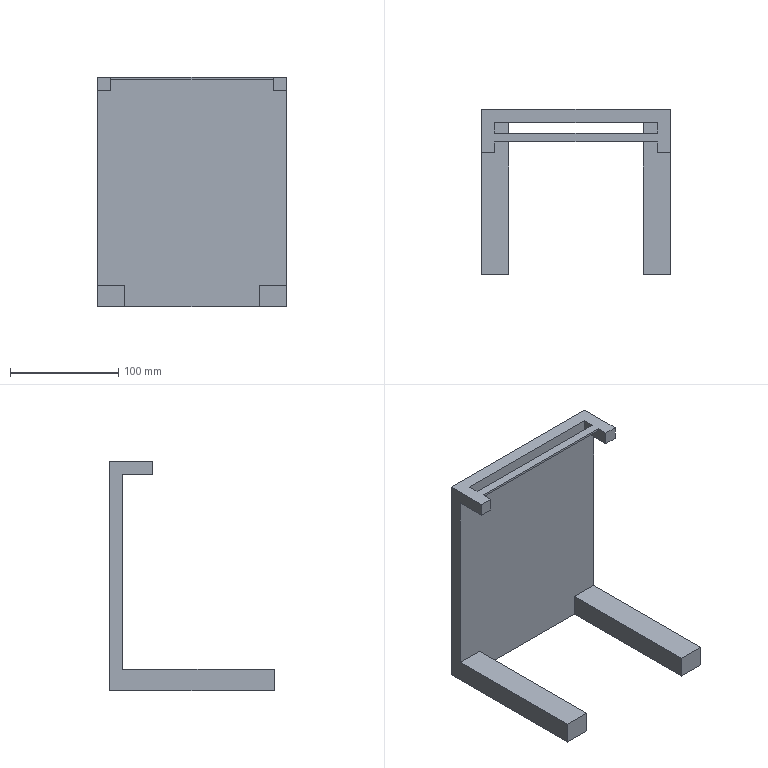Component | SolidWorks | SupportFrame-1 | 1 solid | 21 faces | box 174 x 152 x 212 mm | volume 593120 mm3 | plane 21
build123d program:
from build123d import *

# Parameters (mm, degrees)
SKETCH1_W             = 12
SKETCH1_H             = 12
BOSS_EXTRUDE1_DEPTH   = 40
BOSS_EXTRUDE1_2_DEPTH = 40
SKETCH2_W             = 12
SKETCH2_H             = 12
BOSS_EXTRUDE2_DEPTH   = 150
SKETCH3_W             = 150
SKETCH3_H             = 8
BOSS_EXTRUDE3_DEPTH   = 2
SKETCH4_W             = 174
SKETCH4_H             = 12
BOSS_EXTRUDE4_DEPTH   = 200
SKETCH5_W             = 25
SKETCH5_H             = 20
BOSS_EXTRUDE5_DEPTH   = 140


with BuildPart() as part:
    # Sketch1 → Boss-Extrude1 (new body)
    with BuildSketch(Plane.XY):
        with Locations((-299.265, -73.947)):
            Rectangle(SKETCH1_W, SKETCH1_H)
    extrude(amount=BOSS_EXTRUDE1_DEPTH)



with BuildPart() as body_2:
    # Sketch1 → Boss-Extrude1 2 (new body)
    with BuildSketch(Plane.XY):
        with Locations((-137.265, -73.947)):
            Rectangle(SKETCH1_W, SKETCH1_H)
    extrude(amount=BOSS_EXTRUDE1_2_DEPTH)


with BuildPart() as part_1:
    add(part.part)

    add(body_2.part)  # Boss-Extrude2 merges body 2
    # Sketch2 → Boss-Extrude2 (add)
    with BuildSketch(Plane.ZY.offset(143.265)):
        with Locations((34, -73.947)):
            Rectangle(SKETCH2_W, SKETCH2_H)
    extrude(amount=BOSS_EXTRUDE2_DEPTH)

    # Sketch3 → Boss-Extrude3 (add)
    with BuildSketch(Plane.XZ.offset(79.947)):
        with Locations((-218.265, 14)):
            Rectangle(SKETCH3_W, SKETCH3_H)
    extrude(amount=-BOSS_EXTRUDE3_DEPTH)

    # Sketch4 → Boss-Extrude4 (add)
    with BuildSketch(Plane(origin=(0, -67.947, 0), x_dir=(1, 0, 0), z_dir=(0, 1, 0))):
        with Locations((-218.265, -34)):
            Rectangle(SKETCH4_W, SKETCH4_H)
    extrude(amount=BOSS_EXTRUDE4_DEPTH)

    # Sketch5 → Boss-Extrude5 (add)
    with BuildSketch(Plane(origin=(0, 0, 28), x_dir=(-1, 0, 0), z_dir=(0, 0, -1))):
        with Locations((292.765, 122.053)):
            Rectangle(SKETCH5_W, SKETCH5_H)
        with Locations((143.765, 122.053)):
            Rectangle(SKETCH5_W, SKETCH5_H)
    extrude(amount=BOSS_EXTRUDE5_DEPTH)


solid = part_1.part

# Placed as in the assembly
solid = solid.moved(Location((-81.735, 110, 12.053), (-90, 0, 0)))
STEP:
#1=CARTESIAN_POINT('',(-8.386,5.433,-3.937));
#2=VERTEX_POINT('',#1);
#3=CARTESIAN_POINT('',(-9.37,5.433,-3.937));
#4=VERTEX_POINT('',#3);
#5=CARTESIAN_POINT('',(-8.386,5.433,-3.937));
#6=DIRECTION('',(-1.,0.,0.));
#7=VECTOR('',#6,39.37);
#8=LINE('',#5,#7);
#9=EDGE_CURVE('',#2,#4,#8,.T.);
#10=ORIENTED_EDGE('',*,*,#9,.F.);
#11=CARTESIAN_POINT('',(-8.386,5.433,3.15));
#12=VERTEX_POINT('',#11);
#13=CARTESIAN_POINT('',(-8.386,5.433,-4.724));
#14=DIRECTION('',(0.,0.,1.));
#15=VECTOR('',#14,39.37);
#16=LINE('',#13,#15);
#17=EDGE_CURVE('',#2,#12,#16,.T.);
#18=ORIENTED_EDGE('',*,*,#17,.T.);
#19=CARTESIAN_POINT('',(-8.858,5.433,3.15));
#20=VERTEX_POINT('',#19);
#21=CARTESIAN_POINT('',(-8.386,5.433,3.15));
#22=DIRECTION('',(-1.,0.,0.));
#23=VECTOR('',#22,39.37);
#24=LINE('',#21,#23);
#25=EDGE_CURVE('',#12,#20,#24,.T.);
#26=ORIENTED_EDGE('',*,*,#25,.T.);
#27=CARTESIAN_POINT('',(-8.858,5.433,3.622));
#28=VERTEX_POINT('',#27);
#29=CARTESIAN_POINT('',(-8.858,5.433,3.15));
#30=DIRECTION('',(0.,0.,1.));
#31=VECTOR('',#30,39.37);
#32=LINE('',#29,#31);
#33=EDGE_CURVE('',#20,#28,#32,.T.);
#34=ORIENTED_EDGE('',*,*,#33,.T.);
#35=CARTESIAN_POINT('',(-14.764,5.433,3.622));
#36=VERTEX_POINT('',#35);
#37=CARTESIAN_POINT('',(-15.432,5.433,3.622));
#38=DIRECTION('',(1.,0.,0.));
#39=VECTOR('',#38,39.37);
#40=LINE('',#37,#39);
#41=EDGE_CURVE('',#36,#28,#40,.T.);
#42=ORIENTED_EDGE('',*,*,#41,.F.);
#43=CARTESIAN_POINT('',(-14.764,5.433,3.15));
#44=VERTEX_POINT('',#43);
#45=CARTESIAN_POINT('',(-14.764,5.433,3.15));
#46=DIRECTION('',(0.,0.,1.));
#47=VECTOR('',#46,39.37);
#48=LINE('',#45,#47);
#49=EDGE_CURVE('',#44,#36,#48,.T.);
#50=ORIENTED_EDGE('',*,*,#49,.F.);
#51=CARTESIAN_POINT('',(-15.236,5.433,3.15));
#52=VERTEX_POINT('',#51);
#53=CARTESIAN_POINT('',(-8.386,5.433,3.15));
#54=DIRECTION('',(-1.,0.,0.));
#55=VECTOR('',#54,39.37);
#56=LINE('',#53,#55);
#57=EDGE_CURVE('',#44,#52,#56,.T.);
#58=ORIENTED_EDGE('',*,*,#57,.T.);
#59=CARTESIAN_POINT('',(-15.236,5.433,-3.937));
#60=VERTEX_POINT('',#59);
#61=CARTESIAN_POINT('',(-15.236,5.433,-4.724));
#62=DIRECTION('',(0.,0.,1.));
#63=VECTOR('',#62,39.37);
#64=LINE('',#61,#63);
#65=EDGE_CURVE('',#60,#52,#64,.T.);
#66=ORIENTED_EDGE('',*,*,#65,.F.);
#67=CARTESIAN_POINT('',(-14.252,5.433,-3.937));
#68=VERTEX_POINT('',#67);
#69=CARTESIAN_POINT('',(-15.236,5.433,-3.937));
#70=DIRECTION('',(-1.,0.,0.));
#71=VECTOR('',#70,39.37);
#72=LINE('',#69,#71);
#73=EDGE_CURVE('',#68,#60,#72,.T.);
#74=ORIENTED_EDGE('',*,*,#73,.F.);
#75=CARTESIAN_POINT('',(-14.252,5.433,-4.724));
#76=VERTEX_POINT('',#75);
#77=CARTESIAN_POINT('',(-14.252,5.433,-4.724));
#78=DIRECTION('',(0.,0.,1.));
#79=VECTOR('',#78,39.37);
#80=LINE('',#77,#79);
#81=EDGE_CURVE('',#76,#68,#80,.T.);
#82=ORIENTED_EDGE('',*,*,#81,.F.);
#83=CARTESIAN_POINT('',(-9.37,5.433,-4.724));
#84=VERTEX_POINT('',#83);
#85=CARTESIAN_POINT('',(-8.386,5.433,-4.724));
#86=DIRECTION('',(-1.,0.,0.));
#87=VECTOR('',#86,39.37);
#88=LINE('',#85,#87);
#89=EDGE_CURVE('',#84,#76,#88,.T.);
#90=ORIENTED_EDGE('',*,*,#89,.F.);
#91=CARTESIAN_POINT('',(-9.37,5.433,-4.724));
#92=DIRECTION('',(-0.,-0.,-1.));
#93=VECTOR('',#92,39.37);
#94=LINE('',#91,#93);
#95=EDGE_CURVE('',#4,#84,#94,.T.);
#96=ORIENTED_EDGE('',*,*,#95,.F.);
#97=EDGE_LOOP('',(#10,#18,#26,#34,#42,#50,#58,#66,#74,#82,#90,#96));
#98=FACE_OUTER_BOUND('',#97,.T.);
#99=CARTESIAN_POINT('',(-15.432,5.433,3.15));
#100=DIRECTION('',(0.,1.,-0.));
#101=DIRECTION('',(0.,0.,1.));
#102=AXIS2_PLACEMENT_3D('',#99,#100,#101);
#103=PLANE('',#102);
#104=ADVANCED_FACE('',(#98),#103,.F.);
#105=ORIENTED_EDGE('',*,*,#25,.F.);
#106=CARTESIAN_POINT('',(-8.386,4.331,3.15));
#107=VERTEX_POINT('',#106);
#108=CARTESIAN_POINT('',(-8.386,5.906,3.15));
#109=DIRECTION('',(0.,-1.,0.));
#110=VECTOR('',#109,39.37);
#111=LINE('',#108,#110);
#112=EDGE_CURVE('',#12,#107,#111,.T.);
#113=ORIENTED_EDGE('',*,*,#112,.T.);
#114=CARTESIAN_POINT('',(-8.858,4.331,3.15));
#115=VERTEX_POINT('',#114);
#116=CARTESIAN_POINT('',(-8.858,4.331,3.15));
#117=DIRECTION('',(-1.,0.,0.));
#118=VECTOR('',#117,39.37);
#119=LINE('',#116,#118);
#120=EDGE_CURVE('',#107,#115,#119,.T.);
#121=ORIENTED_EDGE('',*,*,#120,.T.);
#122=CARTESIAN_POINT('',(-8.858,5.906,3.15));
#123=DIRECTION('',(0.,-1.,0.));
#124=VECTOR('',#123,39.37);
#125=LINE('',#122,#124);
#126=EDGE_CURVE('',#20,#115,#125,.T.);
#127=ORIENTED_EDGE('',*,*,#126,.F.);
#128=EDGE_LOOP('',(#105,#113,#121,#127));
#129=FACE_OUTER_BOUND('',#128,.T.);
#130=CARTESIAN_POINT('',(-15.236,5.906,3.15));
#131=DIRECTION('',(0.,0.,1.));
#132=DIRECTION('',(0.,-1.,0.));
#133=AXIS2_PLACEMENT_3D('',#130,#131,#132);
#134=PLANE('',#133);
#135=ADVANCED_FACE('',(#129),#134,.F.);
#136=ORIENTED_EDGE('',*,*,#57,.F.);
#137=CARTESIAN_POINT('',(-14.764,4.331,3.15));
#138=VERTEX_POINT('',#137);
#139=CARTESIAN_POINT('',(-14.764,5.906,3.15));
#140=DIRECTION('',(0.,-1.,0.));
#141=VECTOR('',#140,39.37);
#142=LINE('',#139,#141);
#143=EDGE_CURVE('',#44,#138,#142,.T.);
#144=ORIENTED_EDGE('',*,*,#143,.T.);
#145=CARTESIAN_POINT('',(-15.236,4.331,3.15));
#146=VERTEX_POINT('',#145);
#147=CARTESIAN_POINT('',(-15.236,4.331,3.15));
#148=DIRECTION('',(-1.,0.,0.));
#149=VECTOR('',#148,39.37);
#150=LINE('',#147,#149);
#151=EDGE_CURVE('',#138,#146,#150,.T.);
#152=ORIENTED_EDGE('',*,*,#151,.T.);
#153=CARTESIAN_POINT('',(-15.236,5.906,3.15));
#154=DIRECTION('',(0.,-1.,0.));
#155=VECTOR('',#154,39.37);
#156=LINE('',#153,#155);
#157=EDGE_CURVE('',#52,#146,#156,.T.);
#158=ORIENTED_EDGE('',*,*,#157,.F.);
#159=EDGE_LOOP('',(#136,#144,#152,#158));
#160=FACE_OUTER_BOUND('',#159,.T.);
#161=CARTESIAN_POINT('',(-15.236,5.906,3.15));
#162=DIRECTION('',(0.,0.,1.));
#163=DIRECTION('',(0.,-1.,0.));
#164=AXIS2_PLACEMENT_3D('',#161,#162,#163);
#165=PLANE('',#164);
#166=ADVANCED_FACE('',(#160),#165,.F.);
#167=CARTESIAN_POINT('',(-15.236,4.331,3.622));
#168=VERTEX_POINT('',#167);
#169=CARTESIAN_POINT('',(-15.236,4.331,3.622));
#170=DIRECTION('',(0.,0.,1.));
#171=VECTOR('',#170,39.37);
#172=LINE('',#169,#171);
#173=EDGE_CURVE('',#146,#168,#172,.T.);
#174=ORIENTED_EDGE('',*,*,#173,.T.);
#175=CARTESIAN_POINT('',(-15.236,5.906,3.622));
#176=VERTEX_POINT('',#175);
#177=CARTESIAN_POINT('',(-15.236,5.906,3.622));
#178=DIRECTION('',(0.,-1.,0.));
#179=VECTOR('',#178,39.37);
#180=LINE('',#177,#179);
#181=EDGE_CURVE('',#176,#168,#180,.T.);
#182=ORIENTED_EDGE('',*,*,#181,.F.);
#183=CARTESIAN_POINT('',(-15.236,5.906,-4.724));
#184=VERTEX_POINT('',#183);
#185=CARTESIAN_POINT('',(-15.236,5.906,3.622));
#186=DIRECTION('',(0.,0.,1.));
#187=VECTOR('',#186,39.37);
#188=LINE('',#185,#187);
#189=EDGE_CURVE('',#184,#176,#188,.T.);
#190=ORIENTED_EDGE('',*,*,#189,.F.);
#191=CARTESIAN_POINT('',(-15.236,-0.07874,-4.724));
#192=VERTEX_POINT('',#191);
#193=CARTESIAN_POINT('',(-15.236,5.906,-4.724));
#194=DIRECTION('',(0.,1.,0.));
#195=VECTOR('',#194,39.37);
#196=LINE('',#193,#195);
#197=EDGE_CURVE('',#192,#184,#196,.T.);
#198=ORIENTED_EDGE('',*,*,#197,.F.);
#199=CARTESIAN_POINT('',(-15.236,-0.07874,-3.937));
#200=VERTEX_POINT('',#199);
#201=CARTESIAN_POINT('',(-15.236,-0.07874,-4.724));
#202=DIRECTION('',(0.,-0.,-1.));
#203=VECTOR('',#202,39.37);
#204=LINE('',#201,#203);
#205=EDGE_CURVE('',#200,#192,#204,.T.);
#206=ORIENTED_EDGE('',*,*,#205,.F.);
#207=CARTESIAN_POINT('',(-15.236,-0.07874,-3.937));
#208=DIRECTION('',(0.,1.,-0.));
#209=VECTOR('',#208,39.37);
#210=LINE('',#207,#209);
#211=EDGE_CURVE('',#200,#60,#210,.T.);
#212=ORIENTED_EDGE('',*,*,#211,.T.);
#213=ORIENTED_EDGE('',*,*,#65,.T.);
#214=ORIENTED_EDGE('',*,*,#157,.T.);
#215=EDGE_LOOP('',(#174,#182,#190,#198,#206,#212,#213,#214));
#216=FACE_OUTER_BOUND('',#215,.T.);
#217=CARTESIAN_POINT('',(-15.236,5.906,3.622));
#218=DIRECTION('',(1.,0.,0.));
#219=DIRECTION('',(0.,-1.,0.));
#220=AXIS2_PLACEMENT_3D('',#217,#218,#219);
#221=PLANE('',#220);
#222=ADVANCED_FACE('',(#216),#221,.F.);
#223=CARTESIAN_POINT('',(-14.764,4.724,3.622));
#224=VERTEX_POINT('',#223);
#225=CARTESIAN_POINT('',(-14.764,4.331,3.622));
#226=VERTEX_POINT('',#225);
#227=CARTESIAN_POINT('',(-14.764,5.906,3.622));
#228=DIRECTION('',(0.,-1.,0.));
#229=VECTOR('',#228,39.37);
#230=LINE('',#227,#229);
#231=EDGE_CURVE('',#224,#226,#230,.T.);
#232=ORIENTED_EDGE('',*,*,#231,.F.);
#233=CARTESIAN_POINT('',(-8.858,4.724,3.622));
#234=VERTEX_POINT('',#233);
#235=CARTESIAN_POINT('',(-14.764,4.724,3.622));
#236=DIRECTION('',(1.,0.,0.));
#237=VECTOR('',#236,39.37);
#238=LINE('',#235,#237);
#239=EDGE_CURVE('',#224,#234,#238,.T.);
#240=ORIENTED_EDGE('',*,*,#239,.T.);
#241=CARTESIAN_POINT('',(-8.858,4.331,3.622));
#242=VERTEX_POINT('',#241);
#243=CARTESIAN_POINT('',(-8.858,5.906,3.622));
#244=DIRECTION('',(0.,-1.,0.));
#245=VECTOR('',#244,39.37);
#246=LINE('',#243,#245);
#247=EDGE_CURVE('',#234,#242,#246,.T.);
#248=ORIENTED_EDGE('',*,*,#247,.T.);
#249=CARTESIAN_POINT('',(-8.386,4.331,3.622));
#250=VERTEX_POINT('',#249);
#251=CARTESIAN_POINT('',(-8.858,4.331,3.622));
#252=DIRECTION('',(1.,0.,0.));
#253=VECTOR('',#252,39.37);
#254=LINE('',#251,#253);
#255=EDGE_CURVE('',#242,#250,#254,.T.);
#256=ORIENTED_EDGE('',*,*,#255,.T.);
#257=CARTESIAN_POINT('',(-8.386,5.906,3.622));
#258=VERTEX_POINT('',#257);
#259=CARTESIAN_POINT('',(-8.386,5.906,3.622));
#260=DIRECTION('',(0.,-1.,0.));
#261=VECTOR('',#260,39.37);
#262=LINE('',#259,#261);
#263=EDGE_CURVE('',#258,#250,#262,.T.);
#264=ORIENTED_EDGE('',*,*,#263,.F.);
#265=CARTESIAN_POINT('',(-15.236,5.906,3.622));
#266=DIRECTION('',(1.,0.,0.));
#267=VECTOR('',#266,39.37);
#268=LINE('',#265,#267);
#269=EDGE_CURVE('',#176,#258,#268,.T.);
#270=ORIENTED_EDGE('',*,*,#269,.F.);
#271=ORIENTED_EDGE('',*,*,#181,.T.);
#272=CARTESIAN_POINT('',(-15.236,4.331,3.622));
#273=DIRECTION('',(1.,0.,0.));
#274=VECTOR('',#273,39.37);
#275=LINE('',#272,#274);
#276=EDGE_CURVE('',#168,#226,#275,.T.);
#277=ORIENTED_EDGE('',*,*,#276,.T.);
#278=EDGE_LOOP('',(#232,#240,#248,#256,#264,#270,#271,#277));
#279=FACE_OUTER_BOUND('',#278,.T.);
#280=CARTESIAN_POINT('',(-8.858,5.039,3.622));
#281=VERTEX_POINT('',#280);
#282=CARTESIAN_POINT('',(-14.764,5.039,3.622));
#283=VERTEX_POINT('',#282);
#284=CARTESIAN_POINT('',(-14.764,5.039,3.622));
#285=DIRECTION('',(-1.,0.,0.));
#286=VECTOR('',#285,39.37);
#287=LINE('',#284,#286);
#288=EDGE_CURVE('',#281,#283,#287,.T.);
#289=ORIENTED_EDGE('',*,*,#288,.T.);
#290=CARTESIAN_POINT('',(-14.764,5.906,3.622));
#291=DIRECTION('',(0.,-1.,0.));
#292=VECTOR('',#291,39.37);
#293=LINE('',#290,#292);
#294=EDGE_CURVE('',#36,#283,#293,.T.);
#295=ORIENTED_EDGE('',*,*,#294,.F.);
#296=ORIENTED_EDGE('',*,*,#41,.T.);
#297=CARTESIAN_POINT('',(-8.858,5.906,3.622));
#298=DIRECTION('',(0.,-1.,0.));
#299=VECTOR('',#298,39.37);
#300=LINE('',#297,#299);
#301=EDGE_CURVE('',#28,#281,#300,.T.);
#302=ORIENTED_EDGE('',*,*,#301,.T.);
#303=EDGE_LOOP('',(#289,#295,#296,#302));
#304=FACE_BOUND('',#303,.T.);
#305=CARTESIAN_POINT('',(-15.236,5.906,3.622));
#306=DIRECTION('',(0.,0.,-1.));
#307=DIRECTION('',(0.,1.,0.));
#308=AXIS2_PLACEMENT_3D('',#305,#306,#307);
#309=PLANE('',#308);
#310=ADVANCED_FACE('',(#279,#304),#309,.F.);
#311=ORIENTED_EDGE('',*,*,#294,.T.);
#312=CARTESIAN_POINT('',(-14.764,5.039,3.543));
#313=VERTEX_POINT('',#312);
#314=CARTESIAN_POINT('',(-14.764,5.039,3.543));
#315=DIRECTION('',(0.,0.,1.));
#316=VECTOR('',#315,39.37);
#317=LINE('',#314,#316);
#318=EDGE_CURVE('',#313,#283,#317,.T.);
#319=ORIENTED_EDGE('',*,*,#318,.F.);
#320=CARTESIAN_POINT('',(-14.764,4.724,3.543));
#321=VERTEX_POINT('',#320);
#322=CARTESIAN_POINT('',(-14.764,5.039,3.543));
#323=DIRECTION('',(0.,-1.,0.));
#324=VECTOR('',#323,39.37);
#325=LINE('',#322,#324);
#326=EDGE_CURVE('',#313,#321,#325,.T.);
#327=ORIENTED_EDGE('',*,*,#326,.T.);
#328=CARTESIAN_POINT('',(-14.764,4.724,3.543));
#329=DIRECTION('',(0.,0.,1.));
#330=VECTOR('',#329,39.37);
#331=LINE('',#328,#330);
#332=EDGE_CURVE('',#321,#224,#331,.T.);
#333=ORIENTED_EDGE('',*,*,#332,.T.);
#334=ORIENTED_EDGE('',*,*,#231,.T.);
#335=CARTESIAN_POINT('',(-14.764,4.331,3.622));
#336=DIRECTION('',(0.,0.,-1.));
#337=VECTOR('',#336,39.37);
#338=LINE('',#335,#337);
#339=EDGE_CURVE('',#226,#138,#338,.T.);
#340=ORIENTED_EDGE('',*,*,#339,.T.);
#341=ORIENTED_EDGE('',*,*,#143,.F.);
#342=ORIENTED_EDGE('',*,*,#49,.T.);
#343=EDGE_LOOP('',(#311,#319,#327,#333,#334,#340,#341,#342));
#344=FACE_OUTER_BOUND('',#343,.T.);
#345=CARTESIAN_POINT('',(-14.764,5.906,3.622));
#346=DIRECTION('',(-1.,0.,0.));
#347=DIRECTION('',(0.,1.,0.));
#348=AXIS2_PLACEMENT_3D('',#345,#346,#347);
#349=PLANE('',#348);
#350=ADVANCED_FACE('',(#344),#349,.F.);
#351=ORIENTED_EDGE('',*,*,#189,.T.);
#352=ORIENTED_EDGE('',*,*,#269,.T.);
#353=CARTESIAN_POINT('',(-8.386,5.906,-4.724));
#354=VERTEX_POINT('',#353);
#355=CARTESIAN_POINT('',(-8.386,5.906,3.622));
#356=DIRECTION('',(0.,0.,-1.));
#357=VECTOR('',#356,39.37);
#358=LINE('',#355,#357);
#359=EDGE_CURVE('',#258,#354,#358,.T.);
#360=ORIENTED_EDGE('',*,*,#359,.T.);
#361=CARTESIAN_POINT('',(-8.386,5.906,-4.724));
#362=DIRECTION('',(1.,0.,0.));
#363=VECTOR('',#362,39.37);
#364=LINE('',#361,#363);
#365=EDGE_CURVE('',#184,#354,#364,.T.);
#366=ORIENTED_EDGE('',*,*,#365,.F.);
#367=EDGE_LOOP('',(#351,#352,#360,#366));
#368=FACE_OUTER_BOUND('',#367,.T.);
#369=CARTESIAN_POINT('',(-3.218,5.906,0.4745));
#370=DIRECTION('',(0.,-1.,0.));
#371=DIRECTION('',(-1.,0.,0.));
#372=AXIS2_PLACEMENT_3D('',#369,#370,#371);
#373=PLANE('',#372);
#374=ADVANCED_FACE('',(#368),#373,.F.);
#375=ORIENTED_EDGE('',*,*,#173,.F.);
#376=ORIENTED_EDGE('',*,*,#151,.F.);
#377=ORIENTED_EDGE('',*,*,#339,.F.);
#378=ORIENTED_EDGE('',*,*,#276,.F.);
#379=EDGE_LOOP('',(#375,#376,#377,#378));
#380=FACE_OUTER_BOUND('',#379,.T.);
#381=CARTESIAN_POINT('',(-3.218,4.331,0.4745));
#382=DIRECTION('',(0.,-1.,0.));
#383=DIRECTION('',(-1.,0.,0.));
#384=AXIS2_PLACEMENT_3D('',#381,#382,#383);
#385=PLANE('',#384);
#386=ADVANCED_FACE('',(#380),#385,.T.);
#387=CARTESIAN_POINT('',(-8.858,4.724,3.543));
#388=VERTEX_POINT('',#387);
#389=CARTESIAN_POINT('',(-8.858,5.039,3.543));
#390=VERTEX_POINT('',#389);
#391=CARTESIAN_POINT('',(-8.858,5.039,3.543));
#392=DIRECTION('',(0.,1.,0.));
#393=VECTOR('',#392,39.37);
#394=LINE('',#391,#393);
#395=EDGE_CURVE('',#388,#390,#394,.T.);
#396=ORIENTED_EDGE('',*,*,#395,.T.);
#397=CARTESIAN_POINT('',(-8.858,5.039,3.543));
#398=DIRECTION('',(0.,0.,1.));
#399=VECTOR('',#398,39.37);
#400=LINE('',#397,#399);
#401=EDGE_CURVE('',#390,#281,#400,.T.);
#402=ORIENTED_EDGE('',*,*,#401,.T.);
#403=ORIENTED_EDGE('',*,*,#301,.F.);
#404=ORIENTED_EDGE('',*,*,#33,.F.);
#405=ORIENTED_EDGE('',*,*,#126,.T.);
#406=CARTESIAN_POINT('',(-8.858,4.331,3.622));
#407=DIRECTION('',(0.,0.,1.));
#408=VECTOR('',#407,39.37);
#409=LINE('',#406,#408);
#410=EDGE_CURVE('',#115,#242,#409,.T.);
#411=ORIENTED_EDGE('',*,*,#410,.T.);
#412=ORIENTED_EDGE('',*,*,#247,.F.);
#413=CARTESIAN_POINT('',(-8.858,4.724,3.543));
#414=DIRECTION('',(0.,0.,1.));
#415=VECTOR('',#414,39.37);
#416=LINE('',#413,#415);
#417=EDGE_CURVE('',#388,#234,#416,.T.);
#418=ORIENTED_EDGE('',*,*,#417,.F.);
#419=EDGE_LOOP('',(#396,#402,#403,#404,#405,#411,#412,#418));
#420=FACE_OUTER_BOUND('',#419,.T.);
#421=CARTESIAN_POINT('',(-8.858,5.906,3.622));
#422=DIRECTION('',(1.,0.,0.));
#423=DIRECTION('',(0.,-1.,0.));
#424=AXIS2_PLACEMENT_3D('',#421,#422,#423);
#425=PLANE('',#424);
#426=ADVANCED_FACE('',(#420),#425,.F.);
#427=CARTESIAN_POINT('',(-8.386,4.331,3.622));
#428=DIRECTION('',(0.,0.,-1.));
#429=VECTOR('',#428,39.37);
#430=LINE('',#427,#429);
#431=EDGE_CURVE('',#250,#107,#430,.T.);
#432=ORIENTED_EDGE('',*,*,#431,.T.);
#433=ORIENTED_EDGE('',*,*,#112,.F.);
#434=ORIENTED_EDGE('',*,*,#17,.F.);
#435=CARTESIAN_POINT('',(-8.386,-0.07874,-3.937));
#436=VERTEX_POINT('',#435);
#437=CARTESIAN_POINT('',(-8.386,-0.07874,-3.937));
#438=DIRECTION('',(0.,1.,-0.));
#439=VECTOR('',#438,39.37);
#440=LINE('',#437,#439);
#441=EDGE_CURVE('',#436,#2,#440,.T.);
#442=ORIENTED_EDGE('',*,*,#441,.F.);
#443=CARTESIAN_POINT('',(-8.386,-0.07874,-4.724));
#444=VERTEX_POINT('',#443);
#445=CARTESIAN_POINT('',(-8.386,-0.07874,-4.724));
#446=DIRECTION('',(0.,0.,1.));
#447=VECTOR('',#446,39.37);
#448=LINE('',#445,#447);
#449=EDGE_CURVE('',#444,#436,#448,.T.);
#450=ORIENTED_EDGE('',*,*,#449,.F.);
#451=CARTESIAN_POINT('',(-8.386,5.906,-4.724));
#452=DIRECTION('',(0.,-1.,0.));
#453=VECTOR('',#452,39.37);
#454=LINE('',#451,#453);
#455=EDGE_CURVE('',#354,#444,#454,.T.);
#456=ORIENTED_EDGE('',*,*,#455,.F.);
#457=ORIENTED_EDGE('',*,*,#359,.F.);
#458=ORIENTED_EDGE('',*,*,#263,.T.);
#459=EDGE_LOOP('',(#432,#433,#434,#442,#450,#456,#457,#458));
#460=FACE_OUTER_BOUND('',#459,.T.);
#461=CARTESIAN_POINT('',(-8.386,5.906,3.622));
#462=DIRECTION('',(-1.,0.,0.));
#463=DIRECTION('',(0.,1.,0.));
#464=AXIS2_PLACEMENT_3D('',#461,#462,#463);
#465=PLANE('',#464);
#466=ADVANCED_FACE('',(#460),#465,.F.);
#467=ORIENTED_EDGE('',*,*,#410,.F.);
#468=ORIENTED_EDGE('',*,*,#120,.F.);
#469=ORIENTED_EDGE('',*,*,#431,.F.);
#470=ORIENTED_EDGE('',*,*,#255,.F.);
#471=EDGE_LOOP('',(#467,#468,#469,#470));
#472=FACE_OUTER_BOUND('',#471,.T.);
#473=CARTESIAN_POINT('',(-3.218,4.331,0.4745));
#474=DIRECTION('',(0.,-1.,0.));
#475=DIRECTION('',(-1.,0.,0.));
#476=AXIS2_PLACEMENT_3D('',#473,#474,#475);
#477=PLANE('',#476);
#478=ADVANCED_FACE('',(#472),#477,.T.);
#479=ORIENTED_EDGE('',*,*,#288,.F.);
#480=ORIENTED_EDGE('',*,*,#401,.F.);
#481=CARTESIAN_POINT('',(-14.764,5.039,3.543));
#482=DIRECTION('',(-1.,0.,0.));
#483=VECTOR('',#482,39.37);
#484=LINE('',#481,#483);
#485=EDGE_CURVE('',#390,#313,#484,.T.);
#486=ORIENTED_EDGE('',*,*,#485,.T.);
#487=ORIENTED_EDGE('',*,*,#318,.T.);
#488=EDGE_LOOP('',(#479,#480,#486,#487));
#489=FACE_OUTER_BOUND('',#488,.T.);
#490=CARTESIAN_POINT('',(-14.764,5.039,3.543));
#491=DIRECTION('',(0.,1.,0.));
#492=DIRECTION('',(1.,0.,0.));
#493=AXIS2_PLACEMENT_3D('',#490,#491,#492);
#494=PLANE('',#493);
#495=ADVANCED_FACE('',(#489),#494,.T.);
#496=ORIENTED_EDGE('',*,*,#239,.F.);
#497=ORIENTED_EDGE('',*,*,#332,.F.);
#498=CARTESIAN_POINT('',(-14.764,4.724,3.543));
#499=DIRECTION('',(1.,0.,0.));
#500=VECTOR('',#499,39.37);
#501=LINE('',#498,#500);
#502=EDGE_CURVE('',#321,#388,#501,.T.);
#503=ORIENTED_EDGE('',*,*,#502,.T.);
#504=ORIENTED_EDGE('',*,*,#417,.T.);
#505=EDGE_LOOP('',(#496,#497,#503,#504));
#506=FACE_OUTER_BOUND('',#505,.T.);
#507=CARTESIAN_POINT('',(-14.764,4.724,3.543));
#508=DIRECTION('',(0.,-1.,0.));
#509=DIRECTION('',(-1.,0.,0.));
#510=AXIS2_PLACEMENT_3D('',#507,#508,#509);
#511=PLANE('',#510);
#512=ADVANCED_FACE('',(#506),#511,.T.);
#513=ORIENTED_EDGE('',*,*,#326,.F.);
#514=ORIENTED_EDGE('',*,*,#485,.F.);
#515=ORIENTED_EDGE('',*,*,#395,.F.);
#516=ORIENTED_EDGE('',*,*,#502,.F.);
#517=EDGE_LOOP('',(#513,#514,#515,#516));
#518=FACE_OUTER_BOUND('',#517,.T.);
#519=CARTESIAN_POINT('',(-3.218,4.331,3.543));
#520=DIRECTION('',(0.,0.,1.));
#521=DIRECTION('',(0.,-1.,0.));
#522=AXIS2_PLACEMENT_3D('',#519,#520,#521);
#523=PLANE('',#522);
#524=ADVANCED_FACE('',(#518),#523,.F.);
#525=ORIENTED_EDGE('',*,*,#455,.T.);
#526=CARTESIAN_POINT('',(-9.37,-0.07874,-4.724));
#527=VERTEX_POINT('',#526);
#528=CARTESIAN_POINT('',(-8.386,-0.07874,-4.724));
#529=DIRECTION('',(1.,0.,0.));
#530=VECTOR('',#529,39.37);
#531=LINE('',#528,#530);
#532=EDGE_CURVE('',#527,#444,#531,.T.);
#533=ORIENTED_EDGE('',*,*,#532,.F.);
#534=CARTESIAN_POINT('',(-9.37,-0.07874,-4.724));
#535=DIRECTION('',(0.,1.,-0.));
#536=VECTOR('',#535,39.37);
#537=LINE('',#534,#536);
#538=EDGE_CURVE('',#527,#84,#537,.T.);
#539=ORIENTED_EDGE('',*,*,#538,.T.);
#540=ORIENTED_EDGE('',*,*,#89,.T.);
#541=CARTESIAN_POINT('',(-14.252,-0.07874,-4.724));
#542=VERTEX_POINT('',#541);
#543=CARTESIAN_POINT('',(-14.252,-0.07874,-4.724));
#544=DIRECTION('',(0.,1.,-0.));
#545=VECTOR('',#544,39.37);
#546=LINE('',#543,#545);
#547=EDGE_CURVE('',#542,#76,#546,.T.);
#548=ORIENTED_EDGE('',*,*,#547,.F.);
#549=CARTESIAN_POINT('',(-15.236,-0.07874,-4.724));
#550=DIRECTION('',(1.,0.,0.));
#551=VECTOR('',#550,39.37);
#552=LINE('',#549,#551);
#553=EDGE_CURVE('',#192,#542,#552,.T.);
#554=ORIENTED_EDGE('',*,*,#553,.F.);
#555=ORIENTED_EDGE('',*,*,#197,.T.);
#556=ORIENTED_EDGE('',*,*,#365,.T.);
#557=EDGE_LOOP('',(#525,#533,#539,#540,#548,#554,#555,#556));
#558=FACE_OUTER_BOUND('',#557,.T.);
#559=CARTESIAN_POINT('',(-3.218,4.331,-4.724));
#560=DIRECTION('',(0.,0.,-1.));
#561=DIRECTION('',(0.,1.,0.));
#562=AXIS2_PLACEMENT_3D('',#559,#560,#561);
#563=PLANE('',#562);
#564=ADVANCED_FACE('',(#558),#563,.T.);
#565=ORIENTED_EDGE('',*,*,#81,.T.);
#566=CARTESIAN_POINT('',(-14.252,-0.07874,-3.937));
#567=VERTEX_POINT('',#566);
#568=CARTESIAN_POINT('',(-14.252,-0.07874,-3.937));
#569=DIRECTION('',(0.,1.,-0.));
#570=VECTOR('',#569,39.37);
#571=LINE('',#568,#570);
#572=EDGE_CURVE('',#567,#68,#571,.T.);
#573=ORIENTED_EDGE('',*,*,#572,.F.);
#574=CARTESIAN_POINT('',(-14.252,-0.07874,-4.724));
#575=DIRECTION('',(0.,0.,1.));
#576=VECTOR('',#575,39.37);
#577=LINE('',#574,#576);
#578=EDGE_CURVE('',#542,#567,#577,.T.);
#579=ORIENTED_EDGE('',*,*,#578,.F.);
#580=ORIENTED_EDGE('',*,*,#547,.T.);
#581=EDGE_LOOP('',(#565,#573,#579,#580));
#582=FACE_OUTER_BOUND('',#581,.T.);
#583=CARTESIAN_POINT('',(-14.252,-0.07874,-4.724));
#584=DIRECTION('',(-1.,0.,0.));
#585=DIRECTION('',(0.,1.,0.));
#586=AXIS2_PLACEMENT_3D('',#583,#584,#585);
#587=PLANE('',#586);
#588=ADVANCED_FACE('',(#582),#587,.F.);
#589=ORIENTED_EDGE('',*,*,#73,.T.);
#590=ORIENTED_EDGE('',*,*,#211,.F.);
#591=CARTESIAN_POINT('',(-15.236,-0.07874,-3.937));
#592=DIRECTION('',(-1.,0.,0.));
#593=VECTOR('',#592,39.37);
#594=LINE('',#591,#593);
#595=EDGE_CURVE('',#567,#200,#594,.T.);
#596=ORIENTED_EDGE('',*,*,#595,.F.);
#597=ORIENTED_EDGE('',*,*,#572,.T.);
#598=EDGE_LOOP('',(#589,#590,#596,#597));
#599=FACE_OUTER_BOUND('',#598,.T.);
#600=CARTESIAN_POINT('',(-15.236,-0.07874,-3.937));
#601=DIRECTION('',(0.,-0.,-1.));
#602=DIRECTION('',(0.,1.,-0.));
#603=AXIS2_PLACEMENT_3D('',#600,#601,#602);
#604=PLANE('',#603);
#605=ADVANCED_FACE('',(#599),#604,.F.);
#606=ORIENTED_EDGE('',*,*,#205,.T.);
#607=ORIENTED_EDGE('',*,*,#553,.T.);
#608=ORIENTED_EDGE('',*,*,#578,.T.);
#609=ORIENTED_EDGE('',*,*,#595,.T.);
#610=EDGE_LOOP('',(#606,#607,#608,#609));
#611=FACE_OUTER_BOUND('',#610,.T.);
#612=CARTESIAN_POINT('',(-3.218,-0.07874,0.4745));
#613=DIRECTION('',(0.,1.,-0.));
#614=DIRECTION('',(0.,0.,1.));
#615=AXIS2_PLACEMENT_3D('',#612,#613,#614);
#616=PLANE('',#615);
#617=ADVANCED_FACE('',(#611),#616,.F.);
#618=ORIENTED_EDGE('',*,*,#9,.T.);
#619=CARTESIAN_POINT('',(-9.37,-0.07874,-3.937));
#620=VERTEX_POINT('',#619);
#621=CARTESIAN_POINT('',(-9.37,-0.07874,-3.937));
#622=DIRECTION('',(0.,1.,-0.));
#623=VECTOR('',#622,39.37);
#624=LINE('',#621,#623);
#625=EDGE_CURVE('',#620,#4,#624,.T.);
#626=ORIENTED_EDGE('',*,*,#625,.F.);
#627=CARTESIAN_POINT('',(-8.386,-0.07874,-3.937));
#628=DIRECTION('',(-1.,0.,0.));
#629=VECTOR('',#628,39.37);
#630=LINE('',#627,#629);
#631=EDGE_CURVE('',#436,#620,#630,.T.);
#632=ORIENTED_EDGE('',*,*,#631,.F.);
#633=ORIENTED_EDGE('',*,*,#441,.T.);
#634=EDGE_LOOP('',(#618,#626,#632,#633));
#635=FACE_OUTER_BOUND('',#634,.T.);
#636=CARTESIAN_POINT('',(-8.386,-0.07874,-3.937));
#637=DIRECTION('',(0.,-0.,-1.));
#638=DIRECTION('',(0.,1.,-0.));
#639=AXIS2_PLACEMENT_3D('',#636,#637,#638);
#640=PLANE('',#639);
#641=ADVANCED_FACE('',(#635),#640,.F.);
#642=ORIENTED_EDGE('',*,*,#95,.T.);
#643=ORIENTED_EDGE('',*,*,#538,.F.);
#644=CARTESIAN_POINT('',(-9.37,-0.07874,-4.724));
#645=DIRECTION('',(-0.,-0.,-1.));
#646=VECTOR('',#645,39.37);
#647=LINE('',#644,#646);
#648=EDGE_CURVE('',#620,#527,#647,.T.);
#649=ORIENTED_EDGE('',*,*,#648,.F.);
#650=ORIENTED_EDGE('',*,*,#625,.T.);
#651=EDGE_LOOP('',(#642,#643,#649,#650));
#652=FACE_OUTER_BOUND('',#651,.T.);
#653=CARTESIAN_POINT('',(-9.37,-0.07874,-4.724));
#654=DIRECTION('',(1.,-0.,-0.));
#655=DIRECTION('',(-0.,0.,-1.));
#656=AXIS2_PLACEMENT_3D('',#653,#654,#655);
#657=PLANE('',#656);
#658=ADVANCED_FACE('',(#652),#657,.F.);
#659=ORIENTED_EDGE('',*,*,#449,.T.);
#660=ORIENTED_EDGE('',*,*,#631,.T.);
#661=ORIENTED_EDGE('',*,*,#648,.T.);
#662=ORIENTED_EDGE('',*,*,#532,.T.);
#663=EDGE_LOOP('',(#659,#660,#661,#662));
#664=FACE_OUTER_BOUND('',#663,.T.);
#665=CARTESIAN_POINT('',(-3.218,-0.07874,0.4745));
#666=DIRECTION('',(0.,-1.,0.));
#667=DIRECTION('',(0.,-0.,-1.));
#668=AXIS2_PLACEMENT_3D('',#665,#666,#667);
#669=PLANE('',#668);
#670=ADVANCED_FACE('',(#664),#669,.T.);
#671=CLOSED_SHELL('',(#104,#135,#166,#222,#310,#350,#374,#386,#426,#466,#478,#495,#512,#524,#564,#588,#605,#617,#641,#658,#670));
#672=MANIFOLD_SOLID_BREP('',#671);
#673=CARTESIAN_POINT('',(0.,0.,0.));
#674=DIRECTION('',(0.,0.,1.));
#675=DIRECTION('',(1.,0.,0.));
#676=AXIS2_PLACEMENT_3D('',#673,#674,#675);
#677=(LENGTH_UNIT()NAMED_UNIT(*)SI_UNIT($,.METRE.));
#678=LENGTH_MEASURE_WITH_UNIT(LENGTH_MEASURE(0.0254),#677);
#679=DIMENSIONAL_EXPONENTS(1.,0.,0.,0.,0.,0.,0.);
#680=(CONVERSION_BASED_UNIT('',#678)LENGTH_UNIT()NAMED_UNIT(#679));
#681=UNCERTAINTY_MEASURE_WITH_UNIT(LENGTH_MEASURE(0.00001),#680,'','');
#682=(NAMED_UNIT(*)PLANE_ANGLE_UNIT()SI_UNIT($,.RADIAN.));
#683=(NAMED_UNIT(*)SI_UNIT($,.STERADIAN.)SOLID_ANGLE_UNIT());
#684=(GEOMETRIC_REPRESENTATION_CONTEXT(3)GLOBAL_UNCERTAINTY_ASSIGNED_CONTEXT((#681))GLOBAL_UNIT_ASSIGNED_CONTEXT((#680,#682,#683))REPRESENTATION_CONTEXT('',''));
#685=ADVANCED_BREP_SHAPE_REPRESENTATION('',(#672,#676),#684);
#686=COLOUR_RGB('',0.7922,0.8196,0.9333);
#687=FILL_AREA_STYLE_COLOUR('',#686);
#688=FILL_AREA_STYLE('',(#687));
#689=SURFACE_STYLE_FILL_AREA(#688);
#690=SURFACE_SIDE_STYLE('',(#689));
#691=SURFACE_STYLE_USAGE(.BOTH.,#690);
#692=PRESENTATION_STYLE_ASSIGNMENT((#691));
#693=STYLED_ITEM('',(#692),#672);
#694=(LENGTH_UNIT()NAMED_UNIT(*)SI_UNIT($,.METRE.));
#695=LENGTH_MEASURE_WITH_UNIT(LENGTH_MEASURE(0.0254),#694);
#696=DIMENSIONAL_EXPONENTS(1.,0.,0.,0.,0.,0.,0.);
#697=(CONVERSION_BASED_UNIT('',#695)LENGTH_UNIT()NAMED_UNIT(#696));
#698=UNCERTAINTY_MEASURE_WITH_UNIT(LENGTH_MEASURE(0.00001),#697,'','');
#699=(NAMED_UNIT(*)PLANE_ANGLE_UNIT()SI_UNIT($,.RADIAN.));
#700=(NAMED_UNIT(*)SI_UNIT($,.STERADIAN.)SOLID_ANGLE_UNIT());
#701=(GEOMETRIC_REPRESENTATION_CONTEXT(3)GLOBAL_UNCERTAINTY_ASSIGNED_CONTEXT((#698))GLOBAL_UNIT_ASSIGNED_CONTEXT((#697,#699,#700))REPRESENTATION_CONTEXT('',''));
#702=MECHANICAL_DESIGN_GEOMETRIC_PRESENTATION_REPRESENTATION('',(#693),#701);
#703=PRESENTATION_LAYER_ASSIGNMENT('','',(#693));